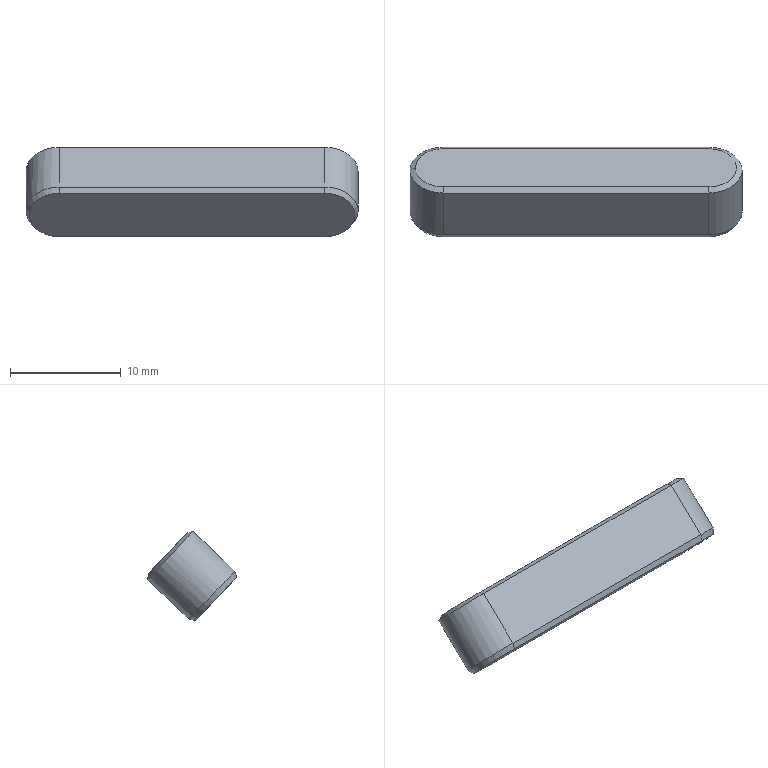Component | SolidWorks | Key6X6-36-1 | 1 solid | 17 faces | box 30 x 8.07 x 8.07 mm | volume 1024 mm3 | plane 8 | cone 6 | cylinder 3 | commonest cylinder face diameters 6 x3 | material Alternative Material
build123d program:
from build123d import *
from OCP.BRepFilletAPI import BRepFilletAPI_MakeChamfer

# Parameters (mm, degrees)
BOSS_EXTRUDE1_DEPTH = 6
CHAMFER1_SIZE       = 0.5
CHAMFER1_SIZE2      = 0.2887


with BuildPart() as part:
    # Sketch1 → Boss-Extrude1 (new body)
    with BuildSketch(Plane.XY):
        with BuildLine():
            Line((-12, 3), (12, 3))
            ThreePointArc((12, 3), (15, 0), (12, -3))
            Line((12, -3), (-12, -3))
            ThreePointArc((-12, -3), (-15, 0), (-12, 3))
        make_face()
    extrude(amount=BOSS_EXTRUDE1_DEPTH)

    # Chamfer1: one chamfer whose edges measure the first distance from different faces: ONE call of the kernel's chamfer builder (chamfer() names one face for all edges)
    chamfer1_edges_1 = [part.edges().sort_by_distance(p)[0] for p in [
        (15, 0, 6),
    ]]
    chamfer1_side_1 = [part.faces().sort_by_distance(p)[0] for p in [
        (15, 0, 3),
    ]]
    chamfer1_edges_2 = [part.edges().sort_by_distance(p)[0] for p in [
        (0, 3, 6),
    ]]
    chamfer1_side_2 = [part.faces().sort_by_distance(p)[0] for p in [
        (0, 3, 3),
    ]]
    chamfer1_edges_3 = [part.edges().sort_by_distance(p)[0] for p in [
        (-15, 0, 6),
    ]]
    chamfer1_side_3 = [part.faces().sort_by_distance(p)[0] for p in [
        (-15, 0, 3),
    ]]
    chamfer1_edges_4 = [part.edges().sort_by_distance(p)[0] for p in [
        (0, 3, 0),
        (15, 0, 0),
        (0, -3, 0),
        (-15, 0, 0),
    ]]
    chamfer1_side_4 = [part.faces().sort_by_distance(p)[0] for p in [
        (0, 0, 0),
    ]]
    chamfer1_edges_5 = [part.edges().sort_by_distance(p)[0] for p in [
        (0, -3, 6),
    ]]
    chamfer1_side_5 = [part.faces().sort_by_distance(p)[0] for p in [
        (0, -3, 3),
    ]]
    chamfer1 = BRepFilletAPI_MakeChamfer(part.part.solid().wrapped)
    for e in chamfer1_edges_1:
        chamfer1.Add(CHAMFER1_SIZE, CHAMFER1_SIZE2, e.wrapped, chamfer1_side_1[0].wrapped)  # the first distance lies on this face
    for e in chamfer1_edges_2:
        chamfer1.Add(CHAMFER1_SIZE, CHAMFER1_SIZE2, e.wrapped, chamfer1_side_2[0].wrapped)  # the first distance lies on this face
    for e in chamfer1_edges_3:
        chamfer1.Add(CHAMFER1_SIZE, CHAMFER1_SIZE2, e.wrapped, chamfer1_side_3[0].wrapped)  # the first distance lies on this face
    for e in chamfer1_edges_4:
        chamfer1.Add(CHAMFER1_SIZE, CHAMFER1_SIZE2, e.wrapped, chamfer1_side_4[0].wrapped)  # the first distance lies on this face
    for e in chamfer1_edges_5:
        chamfer1.Add(CHAMFER1_SIZE, CHAMFER1_SIZE2, e.wrapped, chamfer1_side_5[0].wrapped)  # the first distance lies on this face
    add(Compound.cast(chamfer1.Shape()), mode=Mode.REPLACE)


solid = part.part

# Placed as in the assembly
solid = solid.moved(Location((10.41, -37.957, -24.791), (133.57, 0, 180)))
STEP:
#1=CARTESIAN_POINT('',(0.989,-1.666,-1.139));
#2=VERTEX_POINT('',#1);
#3=CARTESIAN_POINT('',(0.8823,-1.739,-1.062));
#4=VERTEX_POINT('',#3);
#5=CARTESIAN_POINT('',(0.8823,-1.666,-1.139));
#6=DIRECTION('',(0.,-0.7245,-0.6892));
#7=DIRECTION('',(-1.,0.,-0.));
#8=AXIS2_PLACEMENT_3D('',#5,#6,#7);
#9=CIRCLE('',#8,0.1067);
#10=EDGE_CURVE('',#2,#4,#9,.T.);
#11=ORIENTED_EDGE('',*,*,#10,.F.);
#12=CARTESIAN_POINT('',(1.,-1.651,-1.125));
#13=VERTEX_POINT('',#12);
#14=CARTESIAN_POINT('',(0.989,-1.666,-1.139));
#15=DIRECTION('',(0.5,0.6275,0.5969));
#16=VECTOR('',#15,39.37);
#17=LINE('',#14,#16);
#18=EDGE_CURVE('',#2,#13,#17,.T.);
#19=ORIENTED_EDGE('',*,*,#18,.T.);
#20=CARTESIAN_POINT('',(0.8823,-1.733,-1.04));
#21=VERTEX_POINT('',#20);
#22=CARTESIAN_POINT('',(0.8823,-1.651,-1.125));
#23=DIRECTION('',(-0.,0.7245,0.6892));
#24=DIRECTION('',(-1.,0.,-0.));
#25=AXIS2_PLACEMENT_3D('',#22,#23,#24);
#26=CIRCLE('',#25,0.1181);
#27=EDGE_CURVE('',#21,#13,#26,.T.);
#28=ORIENTED_EDGE('',*,*,#27,.F.);
#29=CARTESIAN_POINT('',(0.8823,-1.733,-1.04));
#30=DIRECTION('',(0.,-0.2828,-0.9592));
#31=VECTOR('',#30,39.37);
#32=LINE('',#29,#31);
#33=EDGE_CURVE('',#21,#4,#32,.T.);
#34=ORIENTED_EDGE('',*,*,#33,.T.);
#35=EDGE_LOOP('',(#11,#19,#28,#34));
#36=FACE_OUTER_BOUND('',#35,.T.);
#37=CARTESIAN_POINT('',(0.8823,-1.666,-1.139));
#38=DIRECTION('',(-0.,0.7245,0.6892));
#39=DIRECTION('',(1.,-0.,0.));
#40=AXIS2_PLACEMENT_3D('',#37,#38,#39);
#41=CONICAL_SURFACE('',#40,0.1067,0.5236);
#42=ADVANCED_FACE('',(#36),#41,.T.);
#43=CARTESIAN_POINT('',(-0.161,-1.494,-0.976));
#44=VERTEX_POINT('',#43);
#45=CARTESIAN_POINT('',(-0.06261,-1.562,-0.9047));
#46=VERTEX_POINT('',#45);
#47=CARTESIAN_POINT('',(-0.06261,-1.494,-0.976));
#48=DIRECTION('',(-0.,0.7245,0.6892));
#49=DIRECTION('',(-1.,0.,0.));
#50=AXIS2_PLACEMENT_3D('',#47,#48,#49);
#51=CIRCLE('',#50,0.09843);
#52=EDGE_CURVE('',#44,#46,#51,.T.);
#53=ORIENTED_EDGE('',*,*,#52,.F.);
#54=CARTESIAN_POINT('',(-0.1807,-1.503,-0.9839));
#55=VERTEX_POINT('',#54);
#56=CARTESIAN_POINT('',(-0.1807,-1.503,-0.9839));
#57=DIRECTION('',(-0.866,-0.3623,-0.3446));
#58=VECTOR('',#57,39.37);
#59=LINE('',#56,#58);
#60=EDGE_CURVE('',#44,#55,#59,.T.);
#61=ORIENTED_EDGE('',*,*,#60,.T.);
#62=CARTESIAN_POINT('',(-0.06261,-1.584,-0.8983));
#63=VERTEX_POINT('',#62);
#64=CARTESIAN_POINT('',(-0.06261,-1.503,-0.9839));
#65=DIRECTION('',(0.,-0.7245,-0.6892));
#66=DIRECTION('',(-1.,0.,-0.));
#67=AXIS2_PLACEMENT_3D('',#64,#65,#66);
#68=CIRCLE('',#67,0.1181);
#69=EDGE_CURVE('',#63,#55,#68,.T.);
#70=ORIENTED_EDGE('',*,*,#69,.F.);
#71=CARTESIAN_POINT('',(-0.06261,-1.562,-0.9047));
#72=DIRECTION('',(-0.,-0.9592,0.2828));
#73=VECTOR('',#72,39.37);
#74=LINE('',#71,#73);
#75=EDGE_CURVE('',#46,#63,#74,.T.);
#76=ORIENTED_EDGE('',*,*,#75,.F.);
#77=EDGE_LOOP('',(#53,#61,#70,#76));
#78=FACE_OUTER_BOUND('',#77,.T.);
#79=CARTESIAN_POINT('',(-0.06261,-1.503,-0.9839));
#80=DIRECTION('',(0.,-0.7245,-0.6892));
#81=DIRECTION('',(-1.,0.,-0.));
#82=AXIS2_PLACEMENT_3D('',#79,#80,#81);
#83=CONICAL_SURFACE('',#82,0.1181,1.047);
#84=ADVANCED_FACE('',(#78),#83,.T.);
#85=ORIENTED_EDGE('',*,*,#27,.T.);
#86=CARTESIAN_POINT('',(1.,-1.503,-0.9839));
#87=VERTEX_POINT('',#86);
#88=CARTESIAN_POINT('',(1.,-1.666,-1.139));
#89=DIRECTION('',(-0.,0.7245,0.6892));
#90=VECTOR('',#89,39.37);
#91=LINE('',#88,#90);
#92=EDGE_CURVE('',#13,#87,#91,.T.);
#93=ORIENTED_EDGE('',*,*,#92,.T.);
#94=CARTESIAN_POINT('',(0.8823,-1.584,-0.8983));
#95=VERTEX_POINT('',#94);
#96=CARTESIAN_POINT('',(0.8823,-1.503,-0.9839));
#97=DIRECTION('',(0.,-0.7245,-0.6892));
#98=DIRECTION('',(-1.,0.,-0.));
#99=AXIS2_PLACEMENT_3D('',#96,#97,#98);
#100=CIRCLE('',#99,0.1181);
#101=EDGE_CURVE('',#87,#95,#100,.T.);
#102=ORIENTED_EDGE('',*,*,#101,.T.);
#103=CARTESIAN_POINT('',(0.8823,-1.747,-1.053));
#104=DIRECTION('',(-0.,0.7245,0.6892));
#105=VECTOR('',#104,39.37);
#106=LINE('',#103,#105);
#107=EDGE_CURVE('',#21,#95,#106,.T.);
#108=ORIENTED_EDGE('',*,*,#107,.F.);
#109=EDGE_LOOP('',(#85,#93,#102,#108));
#110=FACE_OUTER_BOUND('',#109,.T.);
#111=CARTESIAN_POINT('',(0.8823,-1.666,-1.139));
#112=DIRECTION('',(-0.,0.7245,0.6892));
#113=DIRECTION('',(1.,-0.,0.));
#114=AXIS2_PLACEMENT_3D('',#111,#112,#113);
#115=CYLINDRICAL_SURFACE('',#114,0.1181);
#116=ADVANCED_FACE('',(#110),#115,.T.);
#117=ORIENTED_EDGE('',*,*,#92,.F.);
#118=CARTESIAN_POINT('',(0.8823,-1.57,-1.211));
#119=VERTEX_POINT('',#118);
#120=CARTESIAN_POINT('',(0.8823,-1.651,-1.125));
#121=DIRECTION('',(-0.,0.7245,0.6892));
#122=DIRECTION('',(-1.,0.,-0.));
#123=AXIS2_PLACEMENT_3D('',#120,#121,#122);
#124=CIRCLE('',#123,0.1181);
#125=EDGE_CURVE('',#13,#119,#124,.T.);
#126=ORIENTED_EDGE('',*,*,#125,.T.);
#127=CARTESIAN_POINT('',(0.8823,-1.421,-1.069));
#128=VERTEX_POINT('',#127);
#129=CARTESIAN_POINT('',(0.8823,-1.584,-1.224));
#130=DIRECTION('',(-0.,0.7245,0.6892));
#131=VECTOR('',#130,39.37);
#132=LINE('',#129,#131);
#133=EDGE_CURVE('',#119,#128,#132,.T.);
#134=ORIENTED_EDGE('',*,*,#133,.T.);
#135=CARTESIAN_POINT('',(0.8823,-1.503,-0.9839));
#136=DIRECTION('',(0.,-0.7245,-0.6892));
#137=DIRECTION('',(-1.,0.,-0.));
#138=AXIS2_PLACEMENT_3D('',#135,#136,#137);
#139=CIRCLE('',#138,0.1181);
#140=EDGE_CURVE('',#128,#87,#139,.T.);
#141=ORIENTED_EDGE('',*,*,#140,.T.);
#142=EDGE_LOOP('',(#117,#126,#134,#141));
#143=FACE_OUTER_BOUND('',#142,.T.);
#144=CARTESIAN_POINT('',(0.8823,-1.666,-1.139));
#145=DIRECTION('',(-0.,0.7245,0.6892));
#146=DIRECTION('',(1.,-0.,0.));
#147=AXIS2_PLACEMENT_3D('',#144,#145,#146);
#148=CYLINDRICAL_SURFACE('',#147,0.1181);
#149=ADVANCED_FACE('',(#143),#148,.T.);
#150=ORIENTED_EDGE('',*,*,#107,.T.);
#151=CARTESIAN_POINT('',(0.8823,-1.584,-0.8983));
#152=DIRECTION('',(-1.,0.,-0.));
#153=VECTOR('',#152,39.37);
#154=LINE('',#151,#153);
#155=EDGE_CURVE('',#95,#63,#154,.T.);
#156=ORIENTED_EDGE('',*,*,#155,.T.);
#157=CARTESIAN_POINT('',(-0.06261,-1.733,-1.04));
#158=VERTEX_POINT('',#157);
#159=CARTESIAN_POINT('',(-0.06261,-1.747,-1.053));
#160=DIRECTION('',(-0.,0.7245,0.6892));
#161=VECTOR('',#160,39.37);
#162=LINE('',#159,#161);
#163=EDGE_CURVE('',#158,#63,#162,.T.);
#164=ORIENTED_EDGE('',*,*,#163,.F.);
#165=CARTESIAN_POINT('',(0.8823,-1.733,-1.04));
#166=DIRECTION('',(1.,-0.,0.));
#167=VECTOR('',#166,39.37);
#168=LINE('',#165,#167);
#169=EDGE_CURVE('',#158,#21,#168,.T.);
#170=ORIENTED_EDGE('',*,*,#169,.T.);
#171=EDGE_LOOP('',(#150,#156,#164,#170));
#172=FACE_OUTER_BOUND('',#171,.T.);
#173=CARTESIAN_POINT('',(0.8823,-1.747,-1.053));
#174=DIRECTION('',(0.,0.6892,-0.7245));
#175=DIRECTION('',(1.,-0.,0.));
#176=AXIS2_PLACEMENT_3D('',#173,#174,#175);
#177=PLANE('',#176);
#178=ADVANCED_FACE('',(#172),#177,.F.);
#179=ORIENTED_EDGE('',*,*,#163,.T.);
#180=ORIENTED_EDGE('',*,*,#69,.T.);
#181=CARTESIAN_POINT('',(-0.06261,-1.421,-1.069));
#182=VERTEX_POINT('',#181);
#183=CARTESIAN_POINT('',(-0.06261,-1.503,-0.9839));
#184=DIRECTION('',(0.,-0.7245,-0.6892));
#185=DIRECTION('',(-1.,0.,-0.));
#186=AXIS2_PLACEMENT_3D('',#183,#184,#185);
#187=CIRCLE('',#186,0.1181);
#188=EDGE_CURVE('',#55,#182,#187,.T.);
#189=ORIENTED_EDGE('',*,*,#188,.T.);
#190=CARTESIAN_POINT('',(-0.06261,-1.57,-1.211));
#191=VERTEX_POINT('',#190);
#192=CARTESIAN_POINT('',(-0.06261,-1.584,-1.224));
#193=DIRECTION('',(-0.,0.7245,0.6892));
#194=VECTOR('',#193,39.37);
#195=LINE('',#192,#194);
#196=EDGE_CURVE('',#191,#182,#195,.T.);
#197=ORIENTED_EDGE('',*,*,#196,.F.);
#198=CARTESIAN_POINT('',(-0.06261,-1.651,-1.125));
#199=DIRECTION('',(-0.,0.7245,0.6892));
#200=DIRECTION('',(-1.,0.,-0.));
#201=AXIS2_PLACEMENT_3D('',#198,#199,#200);
#202=CIRCLE('',#201,0.1181);
#203=EDGE_CURVE('',#191,#158,#202,.T.);
#204=ORIENTED_EDGE('',*,*,#203,.T.);
#205=EDGE_LOOP('',(#179,#180,#189,#197,#204));
#206=FACE_OUTER_BOUND('',#205,.T.);
#207=CARTESIAN_POINT('',(-0.06261,-1.666,-1.139));
#208=DIRECTION('',(-0.,0.7245,0.6892));
#209=DIRECTION('',(1.,-0.,0.));
#210=AXIS2_PLACEMENT_3D('',#207,#208,#209);
#211=CYLINDRICAL_SURFACE('',#210,0.1181);
#212=ADVANCED_FACE('',(#206),#211,.T.);
#213=ORIENTED_EDGE('',*,*,#196,.T.);
#214=CARTESIAN_POINT('',(0.8823,-1.421,-1.069));
#215=DIRECTION('',(1.,-0.,0.));
#216=VECTOR('',#215,39.37);
#217=LINE('',#214,#216);
#218=EDGE_CURVE('',#182,#128,#217,.T.);
#219=ORIENTED_EDGE('',*,*,#218,.T.);
#220=ORIENTED_EDGE('',*,*,#133,.F.);
#221=CARTESIAN_POINT('',(-0.06261,-1.57,-1.211));
#222=DIRECTION('',(-1.,0.,-0.));
#223=VECTOR('',#222,39.37);
#224=LINE('',#221,#223);
#225=EDGE_CURVE('',#119,#191,#224,.T.);
#226=ORIENTED_EDGE('',*,*,#225,.T.);
#227=EDGE_LOOP('',(#213,#219,#220,#226));
#228=FACE_OUTER_BOUND('',#227,.T.);
#229=CARTESIAN_POINT('',(0.8823,-1.584,-1.224));
#230=DIRECTION('',(-0.,-0.6892,0.7245));
#231=DIRECTION('',(-1.,0.,-0.));
#232=AXIS2_PLACEMENT_3D('',#229,#230,#231);
#233=PLANE('',#232);
#234=ADVANCED_FACE('',(#228),#233,.F.);
#235=CARTESIAN_POINT('',(-0.06261,-1.739,-1.062));
#236=VERTEX_POINT('',#235);
#237=CARTESIAN_POINT('',(-0.06261,-1.592,-1.216));
#238=VERTEX_POINT('',#237);
#239=CARTESIAN_POINT('',(-0.06261,-1.666,-1.139));
#240=DIRECTION('',(0.,-0.7245,-0.6892));
#241=DIRECTION('',(-1.,0.,-0.));
#242=AXIS2_PLACEMENT_3D('',#239,#240,#241);
#243=CIRCLE('',#242,0.1067);
#244=EDGE_CURVE('',#236,#238,#243,.T.);
#245=ORIENTED_EDGE('',*,*,#244,.T.);
#246=CARTESIAN_POINT('',(0.8823,-1.592,-1.216));
#247=VERTEX_POINT('',#246);
#248=CARTESIAN_POINT('',(0.8823,-1.592,-1.216));
#249=DIRECTION('',(1.,-0.,0.));
#250=VECTOR('',#249,39.37);
#251=LINE('',#248,#250);
#252=EDGE_CURVE('',#238,#247,#251,.T.);
#253=ORIENTED_EDGE('',*,*,#252,.T.);
#254=CARTESIAN_POINT('',(0.8823,-1.666,-1.139));
#255=DIRECTION('',(0.,-0.7245,-0.6892));
#256=DIRECTION('',(-1.,0.,-0.));
#257=AXIS2_PLACEMENT_3D('',#254,#255,#256);
#258=CIRCLE('',#257,0.1067);
#259=EDGE_CURVE('',#247,#2,#258,.T.);
#260=ORIENTED_EDGE('',*,*,#259,.T.);
#261=ORIENTED_EDGE('',*,*,#10,.T.);
#262=CARTESIAN_POINT('',(-0.06261,-1.739,-1.062));
#263=DIRECTION('',(-1.,0.,-0.));
#264=VECTOR('',#263,39.37);
#265=LINE('',#262,#264);
#266=EDGE_CURVE('',#4,#236,#265,.T.);
#267=ORIENTED_EDGE('',*,*,#266,.T.);
#268=EDGE_LOOP('',(#245,#253,#260,#261,#267));
#269=FACE_OUTER_BOUND('',#268,.T.);
#270=CARTESIAN_POINT('',(0.8823,-1.666,-1.139));
#271=DIRECTION('',(0.,-0.7245,-0.6892));
#272=DIRECTION('',(-1.,0.,-0.));
#273=AXIS2_PLACEMENT_3D('',#270,#271,#272);
#274=PLANE('',#273);
#275=ADVANCED_FACE('',(#269),#274,.T.);
#276=CARTESIAN_POINT('',(-0.06261,-1.427,-1.047));
#277=VERTEX_POINT('',#276);
#278=CARTESIAN_POINT('',(-0.06261,-1.494,-0.976));
#279=DIRECTION('',(-0.,0.7245,0.6892));
#280=DIRECTION('',(-1.,-0.,0.));
#281=AXIS2_PLACEMENT_3D('',#278,#279,#280);
#282=CIRCLE('',#281,0.09843);
#283=EDGE_CURVE('',#277,#44,#282,.T.);
#284=ORIENTED_EDGE('',*,*,#283,.T.);
#285=ORIENTED_EDGE('',*,*,#52,.T.);
#286=CARTESIAN_POINT('',(0.8823,-1.562,-0.9047));
#287=VERTEX_POINT('',#286);
#288=CARTESIAN_POINT('',(0.8823,-1.562,-0.9047));
#289=DIRECTION('',(1.,-0.,0.));
#290=VECTOR('',#289,39.37);
#291=LINE('',#288,#290);
#292=EDGE_CURVE('',#46,#287,#291,.T.);
#293=ORIENTED_EDGE('',*,*,#292,.T.);
#294=CARTESIAN_POINT('',(0.8823,-1.427,-1.047));
#295=VERTEX_POINT('',#294);
#296=CARTESIAN_POINT('',(0.8823,-1.494,-0.976));
#297=DIRECTION('',(-0.,0.7245,0.6892));
#298=DIRECTION('',(-1.,0.,-0.));
#299=AXIS2_PLACEMENT_3D('',#296,#297,#298);
#300=CIRCLE('',#299,0.09843);
#301=EDGE_CURVE('',#287,#295,#300,.T.);
#302=ORIENTED_EDGE('',*,*,#301,.T.);
#303=CARTESIAN_POINT('',(0.8823,-1.427,-1.047));
#304=DIRECTION('',(-1.,0.,-0.));
#305=VECTOR('',#304,39.37);
#306=LINE('',#303,#305);
#307=EDGE_CURVE('',#295,#277,#306,.T.);
#308=ORIENTED_EDGE('',*,*,#307,.T.);
#309=EDGE_LOOP('',(#284,#285,#293,#302,#308));
#310=FACE_OUTER_BOUND('',#309,.T.);
#311=CARTESIAN_POINT('',(0.8823,-1.494,-0.976));
#312=DIRECTION('',(0.,-0.7245,-0.6892));
#313=DIRECTION('',(-1.,0.,-0.));
#314=AXIS2_PLACEMENT_3D('',#311,#312,#313);
#315=PLANE('',#314);
#316=ADVANCED_FACE('',(#310),#315,.F.);
#317=CARTESIAN_POINT('',(-0.06261,-1.427,-1.047));
#318=DIRECTION('',(0.,0.2346,-0.9721));
#319=VECTOR('',#318,39.37);
#320=LINE('',#317,#319);
#321=EDGE_CURVE('',#277,#182,#320,.T.);
#322=ORIENTED_EDGE('',*,*,#321,.F.);
#323=ORIENTED_EDGE('',*,*,#307,.F.);
#324=CARTESIAN_POINT('',(0.8823,-1.421,-1.069));
#325=DIRECTION('',(-0.,-0.2346,0.9721));
#326=VECTOR('',#325,39.37);
#327=LINE('',#324,#326);
#328=EDGE_CURVE('',#128,#295,#327,.T.);
#329=ORIENTED_EDGE('',*,*,#328,.F.);
#330=ORIENTED_EDGE('',*,*,#218,.F.);
#331=EDGE_LOOP('',(#322,#323,#329,#330));
#332=FACE_OUTER_BOUND('',#331,.T.);
#333=CARTESIAN_POINT('',(0.8823,-1.421,-1.069));
#334=DIRECTION('',(-0.,-0.9721,-0.2346));
#335=DIRECTION('',(-0.,-0.2346,0.9721));
#336=AXIS2_PLACEMENT_3D('',#333,#334,#335);
#337=PLANE('',#336);
#338=ADVANCED_FACE('',(#332),#337,.F.);
#339=ORIENTED_EDGE('',*,*,#328,.T.);
#340=ORIENTED_EDGE('',*,*,#301,.F.);
#341=CARTESIAN_POINT('',(0.8823,-1.584,-0.8983));
#342=DIRECTION('',(0.,0.9592,-0.2828));
#343=VECTOR('',#342,39.37);
#344=LINE('',#341,#343);
#345=EDGE_CURVE('',#95,#287,#344,.T.);
#346=ORIENTED_EDGE('',*,*,#345,.F.);
#347=ORIENTED_EDGE('',*,*,#101,.F.);
#348=ORIENTED_EDGE('',*,*,#140,.F.);
#349=EDGE_LOOP('',(#339,#340,#346,#347,#348));
#350=FACE_OUTER_BOUND('',#349,.T.);
#351=CARTESIAN_POINT('',(0.8823,-1.503,-0.9839));
#352=DIRECTION('',(0.,-0.7245,-0.6892));
#353=DIRECTION('',(-1.,0.,-0.));
#354=AXIS2_PLACEMENT_3D('',#351,#352,#353);
#355=CONICAL_SURFACE('',#354,0.1181,1.047);
#356=ADVANCED_FACE('',(#350),#355,.T.);
#357=ORIENTED_EDGE('',*,*,#60,.F.);
#358=ORIENTED_EDGE('',*,*,#283,.F.);
#359=ORIENTED_EDGE('',*,*,#321,.T.);
#360=ORIENTED_EDGE('',*,*,#188,.F.);
#361=EDGE_LOOP('',(#357,#358,#359,#360));
#362=FACE_OUTER_BOUND('',#361,.T.);
#363=CARTESIAN_POINT('',(-0.06261,-1.503,-0.9839));
#364=DIRECTION('',(0.,-0.7245,-0.6892));
#365=DIRECTION('',(-1.,0.,-0.));
#366=AXIS2_PLACEMENT_3D('',#363,#364,#365);
#367=CONICAL_SURFACE('',#366,0.1181,1.047);
#368=ADVANCED_FACE('',(#362),#367,.T.);
#369=ORIENTED_EDGE('',*,*,#345,.T.);
#370=ORIENTED_EDGE('',*,*,#292,.F.);
#371=ORIENTED_EDGE('',*,*,#75,.T.);
#372=ORIENTED_EDGE('',*,*,#155,.F.);
#373=EDGE_LOOP('',(#369,#370,#371,#372));
#374=FACE_OUTER_BOUND('',#373,.T.);
#375=CARTESIAN_POINT('',(0.8823,-1.584,-0.8983));
#376=DIRECTION('',(0.,-0.2828,-0.9592));
#377=DIRECTION('',(-0.,-0.9592,0.2828));
#378=AXIS2_PLACEMENT_3D('',#375,#376,#377);
#379=PLANE('',#378);
#380=ADVANCED_FACE('',(#374),#379,.F.);
#381=ORIENTED_EDGE('',*,*,#33,.F.);
#382=ORIENTED_EDGE('',*,*,#169,.F.);
#383=CARTESIAN_POINT('',(-0.06261,-1.739,-1.062));
#384=DIRECTION('',(-0.,0.2828,0.9592));
#385=VECTOR('',#384,39.37);
#386=LINE('',#383,#385);
#387=EDGE_CURVE('',#236,#158,#386,.T.);
#388=ORIENTED_EDGE('',*,*,#387,.F.);
#389=ORIENTED_EDGE('',*,*,#266,.F.);
#390=EDGE_LOOP('',(#381,#382,#388,#389));
#391=FACE_OUTER_BOUND('',#390,.T.);
#392=CARTESIAN_POINT('',(0.8823,-1.739,-1.062));
#393=DIRECTION('',(-0.,-0.9592,0.2828));
#394=DIRECTION('',(-0.,0.2828,0.9592));
#395=AXIS2_PLACEMENT_3D('',#392,#393,#394);
#396=PLANE('',#395);
#397=ADVANCED_FACE('',(#391),#396,.T.);
#398=ORIENTED_EDGE('',*,*,#387,.T.);
#399=ORIENTED_EDGE('',*,*,#203,.F.);
#400=CARTESIAN_POINT('',(-0.06261,-1.592,-1.216));
#401=DIRECTION('',(0.,0.9721,0.2346));
#402=VECTOR('',#401,39.37);
#403=LINE('',#400,#402);
#404=EDGE_CURVE('',#238,#191,#403,.T.);
#405=ORIENTED_EDGE('',*,*,#404,.F.);
#406=ORIENTED_EDGE('',*,*,#244,.F.);
#407=EDGE_LOOP('',(#398,#399,#405,#406));
#408=FACE_OUTER_BOUND('',#407,.T.);
#409=CARTESIAN_POINT('',(-0.06261,-1.666,-1.139));
#410=DIRECTION('',(-0.,0.7245,0.6892));
#411=DIRECTION('',(1.,-0.,0.));
#412=AXIS2_PLACEMENT_3D('',#409,#410,#411);
#413=CONICAL_SURFACE('',#412,0.1067,0.5236);
#414=ADVANCED_FACE('',(#408),#413,.T.);
#415=ORIENTED_EDGE('',*,*,#18,.F.);
#416=ORIENTED_EDGE('',*,*,#259,.F.);
#417=CARTESIAN_POINT('',(0.8823,-1.57,-1.211));
#418=DIRECTION('',(-0.,-0.9721,-0.2346));
#419=VECTOR('',#418,39.37);
#420=LINE('',#417,#419);
#421=EDGE_CURVE('',#119,#247,#420,.T.);
#422=ORIENTED_EDGE('',*,*,#421,.F.);
#423=ORIENTED_EDGE('',*,*,#125,.F.);
#424=EDGE_LOOP('',(#415,#416,#422,#423));
#425=FACE_OUTER_BOUND('',#424,.T.);
#426=CARTESIAN_POINT('',(0.8823,-1.666,-1.139));
#427=DIRECTION('',(-0.,0.7245,0.6892));
#428=DIRECTION('',(1.,-0.,0.));
#429=AXIS2_PLACEMENT_3D('',#426,#427,#428);
#430=CONICAL_SURFACE('',#429,0.1067,0.5236);
#431=ADVANCED_FACE('',(#425),#430,.T.);
#432=ORIENTED_EDGE('',*,*,#404,.T.);
#433=ORIENTED_EDGE('',*,*,#225,.F.);
#434=ORIENTED_EDGE('',*,*,#421,.T.);
#435=ORIENTED_EDGE('',*,*,#252,.F.);
#436=EDGE_LOOP('',(#432,#433,#434,#435));
#437=FACE_OUTER_BOUND('',#436,.T.);
#438=CARTESIAN_POINT('',(0.8823,-1.592,-1.216));
#439=DIRECTION('',(0.,0.2346,-0.9721));
#440=DIRECTION('',(-0.,-0.9721,-0.2346));
#441=AXIS2_PLACEMENT_3D('',#438,#439,#440);
#442=PLANE('',#441);
#443=ADVANCED_FACE('',(#437),#442,.T.);
#444=CLOSED_SHELL('',(#42,#84,#116,#149,#178,#212,#234,#275,#316,#338,#356,#368,#380,#397,#414,#431,#443));
#445=MANIFOLD_SOLID_BREP('',#444);
#446=CARTESIAN_POINT('',(0.,0.,0.));
#447=DIRECTION('',(0.,0.,1.));
#448=DIRECTION('',(1.,0.,0.));
#449=AXIS2_PLACEMENT_3D('',#446,#447,#448);
#450=(LENGTH_UNIT()NAMED_UNIT(*)SI_UNIT($,.METRE.));
#451=LENGTH_MEASURE_WITH_UNIT(LENGTH_MEASURE(0.0254),#450);
#452=DIMENSIONAL_EXPONENTS(1.,0.,0.,0.,0.,0.,0.);
#453=(CONVERSION_BASED_UNIT('',#451)LENGTH_UNIT()NAMED_UNIT(#452));
#454=UNCERTAINTY_MEASURE_WITH_UNIT(LENGTH_MEASURE(0.00001),#453,'','');
#455=(NAMED_UNIT(*)PLANE_ANGLE_UNIT()SI_UNIT($,.RADIAN.));
#456=(NAMED_UNIT(*)SI_UNIT($,.STERADIAN.)SOLID_ANGLE_UNIT());
#457=(GEOMETRIC_REPRESENTATION_CONTEXT(3)GLOBAL_UNCERTAINTY_ASSIGNED_CONTEXT((#454))GLOBAL_UNIT_ASSIGNED_CONTEXT((#453,#455,#456))REPRESENTATION_CONTEXT('',''));
#458=ADVANCED_BREP_SHAPE_REPRESENTATION('',(#445,#449),#457);
#459=COLOUR_RGB('',0.7922,0.8196,0.9333);
#460=FILL_AREA_STYLE_COLOUR('',#459);
#461=FILL_AREA_STYLE('',(#460));
#462=SURFACE_STYLE_FILL_AREA(#461);
#463=SURFACE_SIDE_STYLE('',(#462));
#464=SURFACE_STYLE_USAGE(.BOTH.,#463);
#465=PRESENTATION_STYLE_ASSIGNMENT((#464));
#466=STYLED_ITEM('',(#465),#445);
#467=PRESENTATION_LAYER_ASSIGNMENT('','',(#466));
#468=(LENGTH_UNIT()NAMED_UNIT(*)SI_UNIT($,.METRE.));
#469=LENGTH_MEASURE_WITH_UNIT(LENGTH_MEASURE(0.0254),#468);
#470=DIMENSIONAL_EXPONENTS(1.,0.,0.,0.,0.,0.,0.);
#471=(CONVERSION_BASED_UNIT('',#469)LENGTH_UNIT()NAMED_UNIT(#470));
#472=UNCERTAINTY_MEASURE_WITH_UNIT(LENGTH_MEASURE(0.00001),#471,'','');
#473=(NAMED_UNIT(*)PLANE_ANGLE_UNIT()SI_UNIT($,.RADIAN.));
#474=(NAMED_UNIT(*)SI_UNIT($,.STERADIAN.)SOLID_ANGLE_UNIT());
#475=(GEOMETRIC_REPRESENTATION_CONTEXT(3)GLOBAL_UNCERTAINTY_ASSIGNED_CONTEXT((#472))GLOBAL_UNIT_ASSIGNED_CONTEXT((#471,#473,#474))REPRESENTATION_CONTEXT('',''));
#476=MECHANICAL_DESIGN_GEOMETRIC_PRESENTATION_REPRESENTATION('',(#466),#475);